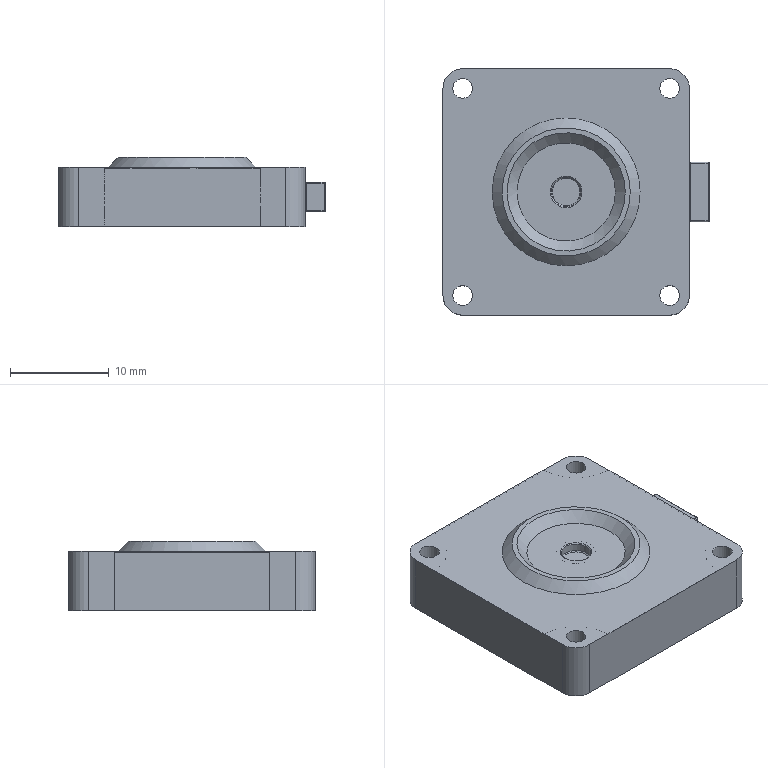Component | NX | STEPPER_BACK | 1 solid | 91 faces | volume 499 mm3 | cylinder 41 | plane 29 | cone 7 | sphere 7 | torus 7 | commonest cylinder face diameters 0.2 x23 4 x5 2 x4 9.2 x4 1 x3 3 x2